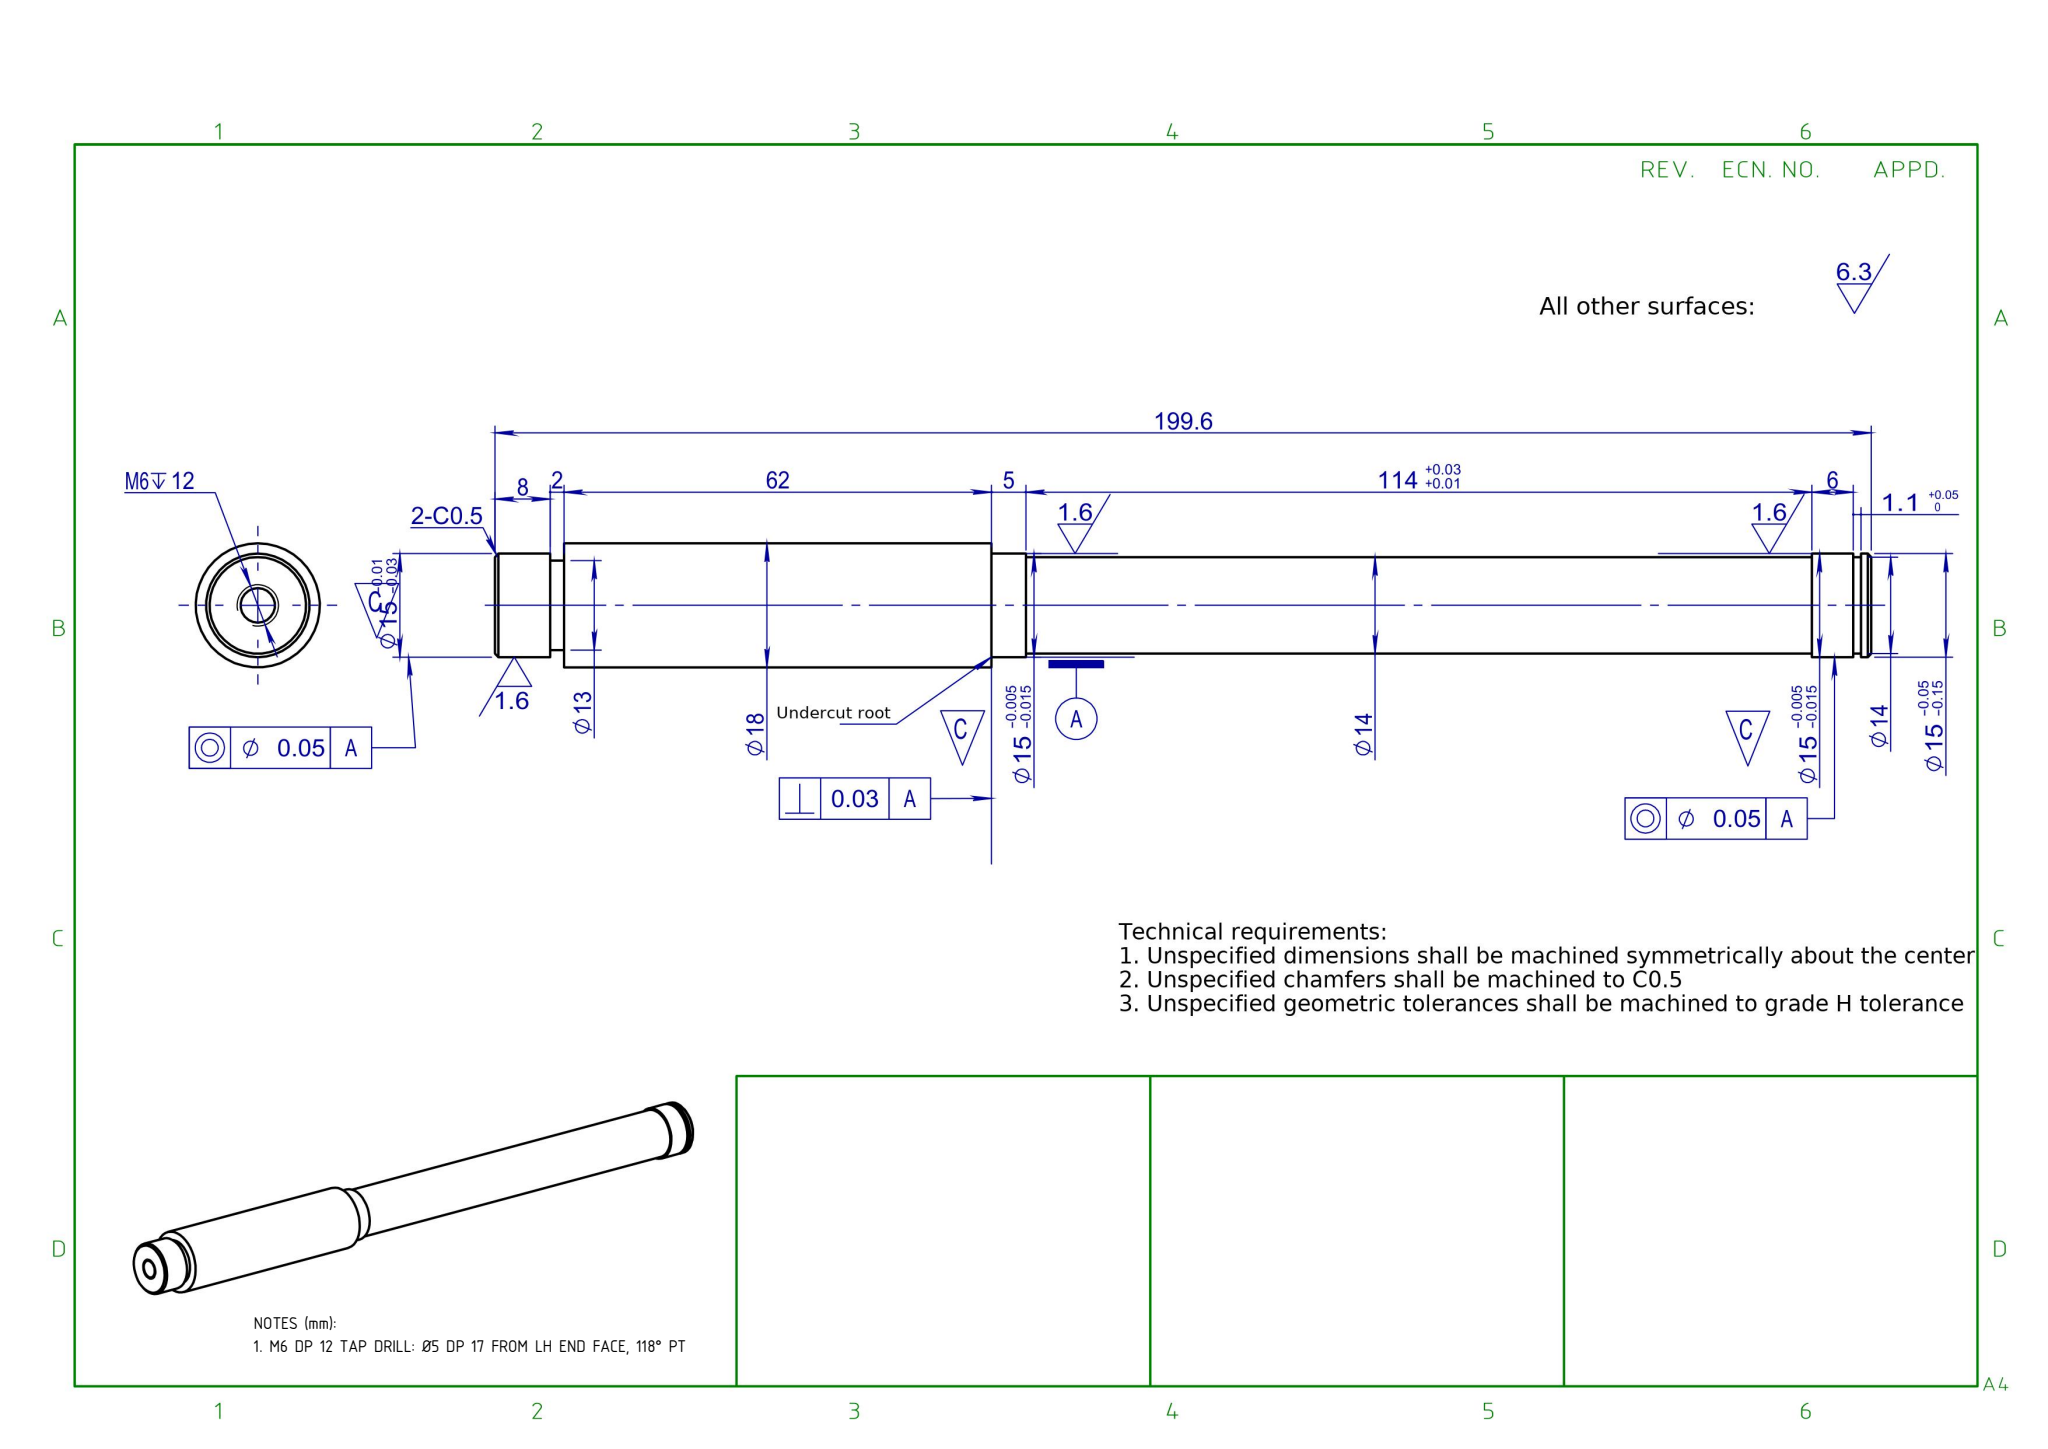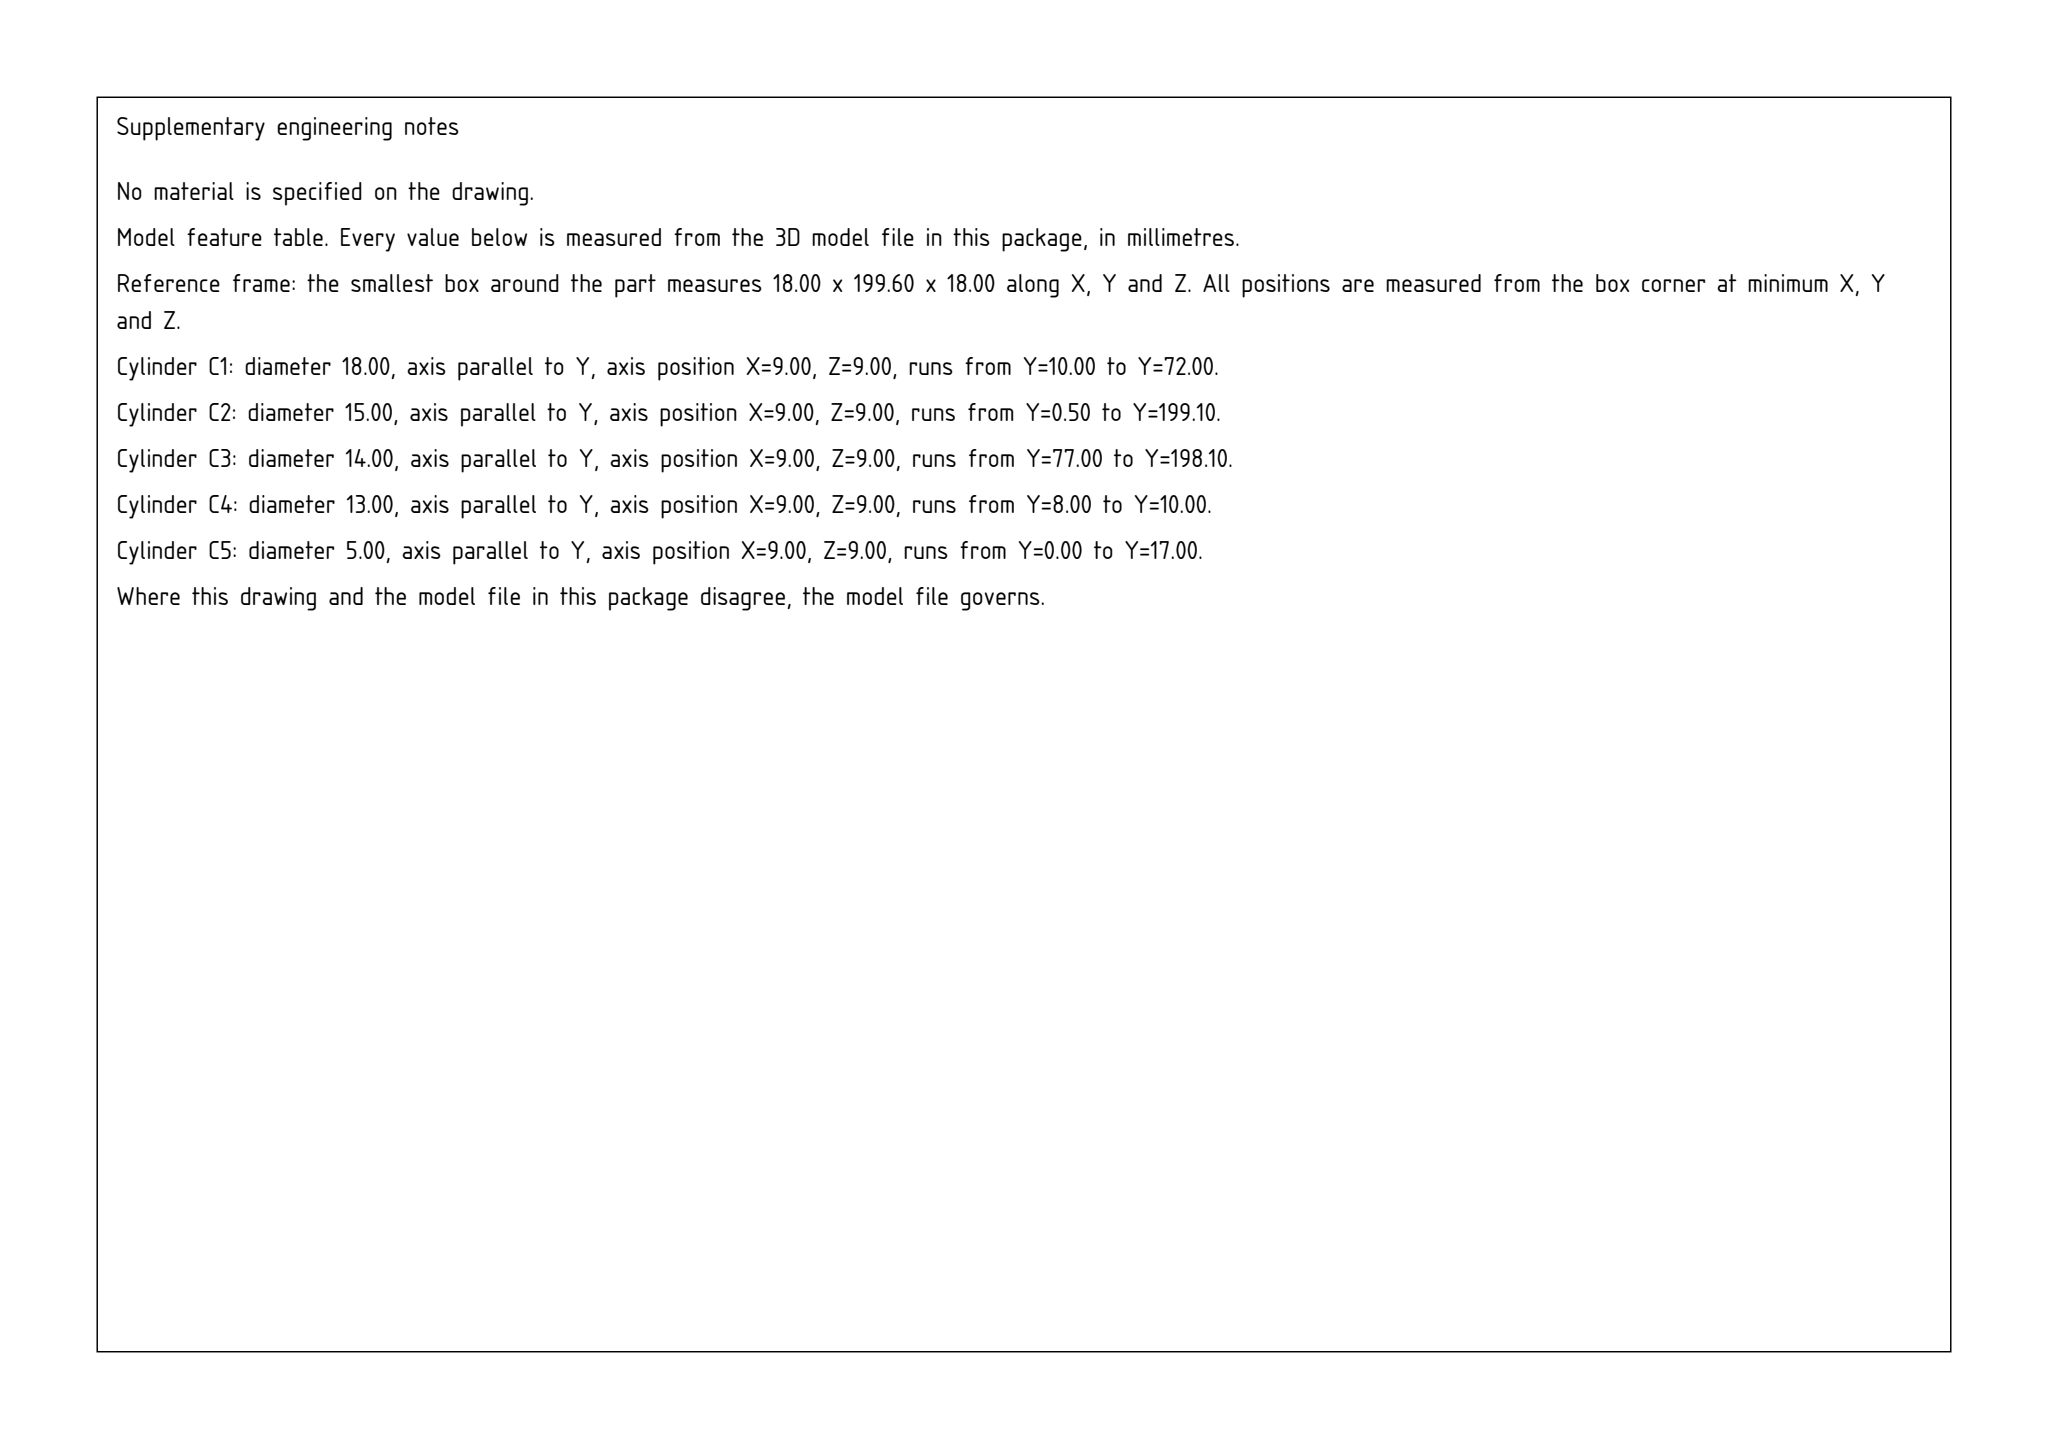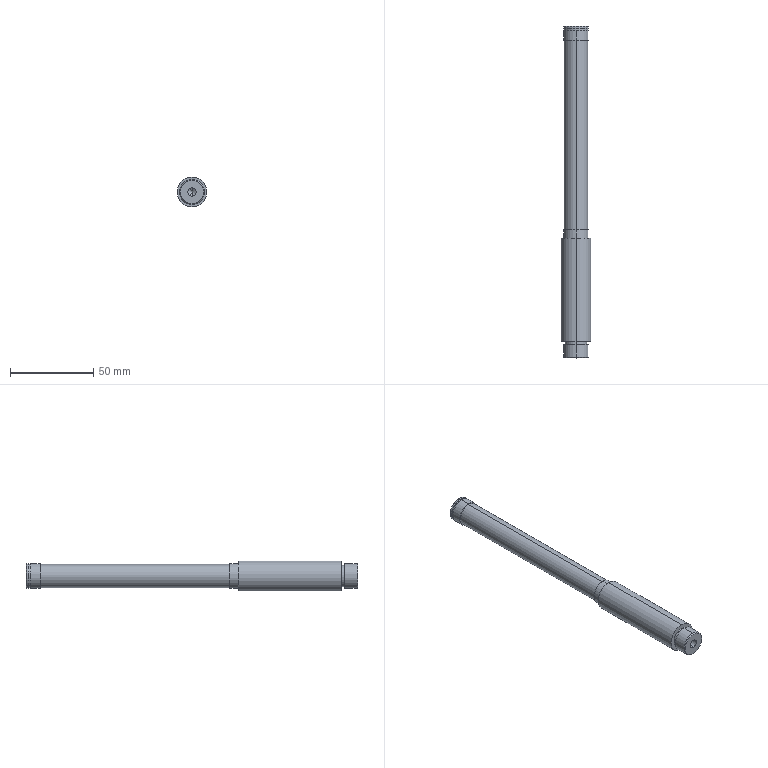Part | SolidWorks | mm | 1 solid | 33 faces | box 18 x 199.6 x 18 mm | volume 37028 mm3 | cylinder 18 | plane 9 | cone 6 | commonest cylinder face diameters 15 x8 14 x4 5 x2 13 x2 18 x2
Drawing notes:
M6 DP 12 TAP DRILL: Ø5 DP 17 FROM LH END FACE, 118° PT | from the solid: cylinder dia 5.0 axis y at (9,9), length 17.0 starting at y=0 end face; cone incl angle 118° ref dia 5.0
build123d program:
from build123d import *

# Parameters (mm, degrees)
SKETCH1_R             = 7.5
EXTRUDE1_DEPTH        = 10
SKETCH2_R             = 9
EXTRUDE2_DEPTH        = 62
SKETCH3_R             = 7.5
EXTRUDE3_DEPTH        = 5
SKETCH4_R             = 7
EXTRUDE4_DEPTH        = 114
SKETCH5_R             = 7.5
EXTRUDE5_DEPTH        = 6
SKETCH6_R             = 7
EXTRUDE6_DEPTH        = 1.1
SKETCH7_R             = 7.5
EXTRUDE7_DEPTH        = 1.5
CHAMFER1_SIZE         = 0.5
M6_TAPPED_HOLE1_D     = 5
M6_TAPPED_HOLE1_DEPTH = 17
M6_TAPPED_HOLE1_TIP   = 1.502
SKETCH10_W            = 1
SKETCH10_H            = 2
CHAMFER2_SIZE         = 0.5


with BuildPart() as part:
    # Sketch1 → Extrude1 (new body)
    with BuildSketch(Plane(origin=(0, 0, 0), x_dir=(1, 0, 0), z_dir=(0, 1, 0))):
        with Locations(Location((0, 0, 0), (0, 0, 270))):
            Circle(SKETCH1_R)
    extrude(amount=EXTRUDE1_DEPTH)

    # Sketch2 → Extrude2 (add)
    with BuildSketch(Plane(origin=(0, 10, 0), x_dir=(1, 0, 0), z_dir=(0, 1, 0))):
        with Locations(Location((0, 0, 0), (0, 0, 270))):
            Circle(SKETCH2_R)
    extrude(amount=EXTRUDE2_DEPTH)

    # Sketch3 → Extrude3 (add)
    with BuildSketch(Plane(origin=(0, 72, 0), x_dir=(1, 0, 0), z_dir=(0, 1, 0))):
        with Locations(Location((0, 0, 0), (0, 0, 270))):
            Circle(SKETCH3_R)
    extrude(amount=EXTRUDE3_DEPTH)

    # Sketch4 → Extrude4 (add)
    with BuildSketch(Plane(origin=(0, 77, 0), x_dir=(1, 0, 0), z_dir=(0, 1, 0))):
        with Locations(Location((0, 0, 0), (0, 0, 90))):
            Circle(SKETCH4_R)
    extrude(amount=EXTRUDE4_DEPTH)

    # Sketch5 → Extrude5 (add)
    with BuildSketch(Plane(origin=(0, 191, 0), x_dir=(1, 0, 0), z_dir=(0, 1, 0))):
        with Locations(Location((0, 0, 0), (0, 0, 270))):
            Circle(SKETCH5_R)
    extrude(amount=EXTRUDE5_DEPTH)

    # Sketch6 → Extrude6 (add)
    with BuildSketch(Plane(origin=(0, 197, 0), x_dir=(1, 0, 0), z_dir=(0, 1, 0))):
        with Locations(Location((0, 0, 0), (0, 0, 90))):
            Circle(SKETCH6_R)
    extrude(amount=EXTRUDE6_DEPTH)

    # Sketch7 → Extrude7 (add)
    with BuildSketch(Plane(origin=(0, 198.1, 0), x_dir=(1, 0, 0), z_dir=(0, 1, 0))):
        with Locations(Location((0, 0, 0), (0, 0, 270))):
            Circle(SKETCH7_R)
    extrude(amount=EXTRUDE7_DEPTH)

    # Chamfer1
    chamfer1_edges = [part.edges().sort_by_distance(p)[0] for p in [
        (0, 199.6, -7.5),
    ]]
    chamfer(chamfer1_edges, length=CHAMFER1_SIZE)

    # M6 Tapped Hole1
    with Locations(Plane.XZ):
        with Locations((0, 0)):
            Hole(M6_TAPPED_HOLE1_D / 2, depth=M6_TAPPED_HOLE1_DEPTH)
            with Locations((0, 0, -(M6_TAPPED_HOLE1_DEPTH + M6_TAPPED_HOLE1_TIP / 2))):  # 118° drill point
                Cone(0, M6_TAPPED_HOLE1_D / 2, M6_TAPPED_HOLE1_TIP, mode=Mode.SUBTRACT)

    # Sketch10 → Revolve-Cut1 (revolve, cut)
    with BuildSketch(Plane.XY, mode=Mode.PRIVATE) as revolve_cut1_sk:
        with Locations((-7, 9)):
            Rectangle(SKETCH10_W, SKETCH10_H)
    revolve(revolve_cut1_sk.sketch.rotate(Axis((0, 0, 0), (0, 1, 0)), 270), axis=Axis((0, 0, 0), (0, 1, 0)), mode=Mode.SUBTRACT)

    # Chamfer2
    chamfer2_edges = [part.edges().sort_by_distance(p)[0] for p in [
        (0, 0, -7.5),
    ]]
    chamfer(chamfer2_edges, length=CHAMFER2_SIZE)


solid = part.part
STEP:
#1=CARTESIAN_POINT('',(0.,0.,-7.));
#2=VERTEX_POINT('',#1);
#3=CARTESIAN_POINT('',(0.,0.,7.));
#4=VERTEX_POINT('',#3);
#5=CARTESIAN_POINT('',(0.,0.,0.));
#6=DIRECTION('',(0.,-1.,0.));
#7=DIRECTION('',(0.,0.,1.));
#8=AXIS2_PLACEMENT_3D('',#5,#6,#7);
#9=CIRCLE('',#8,7.);
#10=EDGE_CURVE('',#2,#4,#9,.T.);
#11=ORIENTED_EDGE('',*,*,#10,.F.);
#12=CARTESIAN_POINT('',(0.,0.5,-7.5));
#13=VERTEX_POINT('',#12);
#14=CARTESIAN_POINT('',(0.,0.5,-7.5));
#15=DIRECTION('',(0.,0.7071,-0.7071));
#16=VECTOR('',#15,1000.);
#17=LINE('',#14,#16);
#18=EDGE_CURVE('',#2,#13,#17,.T.);
#19=ORIENTED_EDGE('',*,*,#18,.T.);
#20=CARTESIAN_POINT('',(0.,0.5,7.5));
#21=VERTEX_POINT('',#20);
#22=CARTESIAN_POINT('',(0.,0.5,0.));
#23=DIRECTION('',(0.,1.,0.));
#24=DIRECTION('',(0.,0.,1.));
#25=AXIS2_PLACEMENT_3D('',#22,#23,#24);
#26=CIRCLE('',#25,7.5);
#27=EDGE_CURVE('',#21,#13,#26,.T.);
#28=ORIENTED_EDGE('',*,*,#27,.F.);
#29=CARTESIAN_POINT('',(0.,0.5,7.5));
#30=DIRECTION('',(0.,0.7071,0.7071));
#31=VECTOR('',#30,1000.);
#32=LINE('',#29,#31);
#33=EDGE_CURVE('',#4,#21,#32,.T.);
#34=ORIENTED_EDGE('',*,*,#33,.F.);
#35=EDGE_LOOP('',(#11,#19,#28,#34));
#36=FACE_OUTER_BOUND('',#35,.T.);
#37=CARTESIAN_POINT('',(0.,0.5,0.));
#38=DIRECTION('',(0.,1.,0.));
#39=DIRECTION('',(0.,0.,1.));
#40=AXIS2_PLACEMENT_3D('',#37,#38,#39);
#41=CONICAL_SURFACE('',#40,7.5,0.7854);
#42=ADVANCED_FACE('',(#36),#41,.T.);
#43=CARTESIAN_POINT('',(0.,8.,-7.5));
#44=VERTEX_POINT('',#43);
#45=CARTESIAN_POINT('',(0.,8.,7.5));
#46=VERTEX_POINT('',#45);
#47=CARTESIAN_POINT('',(0.,8.,0.));
#48=DIRECTION('',(0.,-1.,0.));
#49=DIRECTION('',(0.,0.,-1.));
#50=AXIS2_PLACEMENT_3D('',#47,#48,#49);
#51=CIRCLE('',#50,7.5);
#52=EDGE_CURVE('',#44,#46,#51,.T.);
#53=ORIENTED_EDGE('',*,*,#52,.T.);
#54=CARTESIAN_POINT('',(0.,10.,7.5));
#55=DIRECTION('',(0.,-1.,0.));
#56=VECTOR('',#55,1000.);
#57=LINE('',#54,#56);
#58=EDGE_CURVE('',#46,#21,#57,.T.);
#59=ORIENTED_EDGE('',*,*,#58,.T.);
#60=ORIENTED_EDGE('',*,*,#27,.T.);
#61=CARTESIAN_POINT('',(0.,10.,-7.5));
#62=DIRECTION('',(0.,-1.,0.));
#63=VECTOR('',#62,1000.);
#64=LINE('',#61,#63);
#65=EDGE_CURVE('',#44,#13,#64,.T.);
#66=ORIENTED_EDGE('',*,*,#65,.F.);
#67=EDGE_LOOP('',(#53,#59,#60,#66));
#68=FACE_OUTER_BOUND('',#67,.T.);
#69=CARTESIAN_POINT('',(0.,10.,0.));
#70=DIRECTION('',(0.,-1.,0.));
#71=DIRECTION('',(0.,0.,-1.));
#72=AXIS2_PLACEMENT_3D('',#69,#70,#71);
#73=CYLINDRICAL_SURFACE('',#72,7.5);
#74=ADVANCED_FACE('',(#68),#73,.T.);
#75=CARTESIAN_POINT('',(0.,17.,2.5));
#76=VERTEX_POINT('',#75);
#77=CARTESIAN_POINT('',(0.,17.,-2.5));
#78=VERTEX_POINT('',#77);
#79=CARTESIAN_POINT('',(0.,17.,0.));
#80=DIRECTION('',(0.,-1.,0.));
#81=DIRECTION('',(0.,0.,-1.));
#82=AXIS2_PLACEMENT_3D('',#79,#80,#81);
#83=CIRCLE('',#82,2.5);
#84=EDGE_CURVE('',#76,#78,#83,.T.);
#85=ORIENTED_EDGE('',*,*,#84,.F.);
#86=CARTESIAN_POINT('',(0.,-0.,2.5));
#87=VERTEX_POINT('',#86);
#88=CARTESIAN_POINT('',(0.,0.,2.5));
#89=DIRECTION('',(0.,-1.,0.));
#90=VECTOR('',#89,1000.);
#91=LINE('',#88,#90);
#92=EDGE_CURVE('',#76,#87,#91,.T.);
#93=ORIENTED_EDGE('',*,*,#92,.T.);
#94=CARTESIAN_POINT('',(0.,-0.,-2.5));
#95=VERTEX_POINT('',#94);
#96=CARTESIAN_POINT('',(0.,-0.,0.));
#97=DIRECTION('',(0.,-1.,0.));
#98=DIRECTION('',(0.,0.,-1.));
#99=AXIS2_PLACEMENT_3D('',#96,#97,#98);
#100=CIRCLE('',#99,2.5);
#101=EDGE_CURVE('',#87,#95,#100,.T.);
#102=ORIENTED_EDGE('',*,*,#101,.T.);
#103=CARTESIAN_POINT('',(0.,0.,-2.5));
#104=DIRECTION('',(0.,-1.,0.));
#105=VECTOR('',#104,1000.);
#106=LINE('',#103,#105);
#107=EDGE_CURVE('',#78,#95,#106,.T.);
#108=ORIENTED_EDGE('',*,*,#107,.F.);
#109=EDGE_LOOP('',(#85,#93,#102,#108));
#110=FACE_OUTER_BOUND('',#109,.T.);
#111=CARTESIAN_POINT('',(0.,0.,0.));
#112=DIRECTION('',(0.,-1.,0.));
#113=DIRECTION('',(0.,0.,-1.));
#114=AXIS2_PLACEMENT_3D('',#111,#112,#113);
#115=CYLINDRICAL_SURFACE('',#114,2.5);
#116=ADVANCED_FACE('',(#110),#115,.F.);
#117=CARTESIAN_POINT('',(-0.,18.502,0.));
#118=VERTEX_POINT('',#117);
#119=CARTESIAN_POINT('',(0.,17.,-2.5));
#120=DIRECTION('',(0.,-0.515,-0.8572));
#121=VECTOR('',#120,1000.);
#122=LINE('',#119,#121);
#123=EDGE_CURVE('',#118,#78,#122,.T.);
#124=ORIENTED_EDGE('',*,*,#123,.F.);
#125=CARTESIAN_POINT('',(0.,17.,2.5));
#126=DIRECTION('',(0.,-0.515,0.8572));
#127=VECTOR('',#126,1000.);
#128=LINE('',#125,#127);
#129=EDGE_CURVE('',#118,#76,#128,.T.);
#130=ORIENTED_EDGE('',*,*,#129,.T.);
#131=ORIENTED_EDGE('',*,*,#84,.T.);
#132=EDGE_LOOP('',(#124,#130,#131));
#133=FACE_OUTER_BOUND('',#132,.T.);
#134=CARTESIAN_POINT('',(0.,17.,0.));
#135=DIRECTION('',(0.,-1.,0.));
#136=DIRECTION('',(0.,0.,-1.));
#137=AXIS2_PLACEMENT_3D('',#134,#135,#136);
#138=CONICAL_SURFACE('',#137,2.5,1.03);
#139=ADVANCED_FACE('',(#133),#138,.F.);
#140=CARTESIAN_POINT('',(0.,10.,-6.5));
#141=VERTEX_POINT('',#140);
#142=CARTESIAN_POINT('',(0.,10.,6.5));
#143=VERTEX_POINT('',#142);
#144=CARTESIAN_POINT('',(0.,10.,0.));
#145=DIRECTION('',(0.,-1.,0.));
#146=DIRECTION('',(0.,0.,-1.));
#147=AXIS2_PLACEMENT_3D('',#144,#145,#146);
#148=CIRCLE('',#147,6.5);
#149=EDGE_CURVE('',#141,#143,#148,.T.);
#150=ORIENTED_EDGE('',*,*,#149,.T.);
#151=CARTESIAN_POINT('',(0.,8.,6.5));
#152=VERTEX_POINT('',#151);
#153=CARTESIAN_POINT('',(0.,0.,6.5));
#154=DIRECTION('',(0.,-1.,0.));
#155=VECTOR('',#154,1000.);
#156=LINE('',#153,#155);
#157=EDGE_CURVE('',#143,#152,#156,.T.);
#158=ORIENTED_EDGE('',*,*,#157,.T.);
#159=CARTESIAN_POINT('',(0.,8.,-6.5));
#160=VERTEX_POINT('',#159);
#161=CARTESIAN_POINT('',(0.,8.,0.));
#162=DIRECTION('',(0.,-1.,0.));
#163=DIRECTION('',(0.,0.,-1.));
#164=AXIS2_PLACEMENT_3D('',#161,#162,#163);
#165=CIRCLE('',#164,6.5);
#166=EDGE_CURVE('',#160,#152,#165,.T.);
#167=ORIENTED_EDGE('',*,*,#166,.F.);
#168=CARTESIAN_POINT('',(0.,0.,-6.5));
#169=DIRECTION('',(0.,-1.,0.));
#170=VECTOR('',#169,1000.);
#171=LINE('',#168,#170);
#172=EDGE_CURVE('',#141,#160,#171,.T.);
#173=ORIENTED_EDGE('',*,*,#172,.F.);
#174=EDGE_LOOP('',(#150,#158,#167,#173));
#175=FACE_OUTER_BOUND('',#174,.T.);
#176=CARTESIAN_POINT('',(0.,0.,0.));
#177=DIRECTION('',(0.,-1.,0.));
#178=DIRECTION('',(0.,0.,-1.));
#179=AXIS2_PLACEMENT_3D('',#176,#177,#178);
#180=CYLINDRICAL_SURFACE('',#179,6.5);
#181=ADVANCED_FACE('',(#175),#180,.T.);
#182=CARTESIAN_POINT('',(0.,199.6,7.));
#183=VERTEX_POINT('',#182);
#184=CARTESIAN_POINT('',(0.,199.6,-7.));
#185=VERTEX_POINT('',#184);
#186=CARTESIAN_POINT('',(0.,199.6,0.));
#187=DIRECTION('',(0.,1.,0.));
#188=DIRECTION('',(0.,0.,1.));
#189=AXIS2_PLACEMENT_3D('',#186,#187,#188);
#190=CIRCLE('',#189,7.);
#191=EDGE_CURVE('',#183,#185,#190,.T.);
#192=ORIENTED_EDGE('',*,*,#191,.F.);
#193=CARTESIAN_POINT('',(0.,199.1,7.5));
#194=VERTEX_POINT('',#193);
#195=CARTESIAN_POINT('',(0.,199.6,7.));
#196=DIRECTION('',(0.,-0.7071,0.7071));
#197=VECTOR('',#196,1000.);
#198=LINE('',#195,#197);
#199=EDGE_CURVE('',#183,#194,#198,.T.);
#200=ORIENTED_EDGE('',*,*,#199,.T.);
#201=CARTESIAN_POINT('',(0.,199.1,-7.5));
#202=VERTEX_POINT('',#201);
#203=CARTESIAN_POINT('',(0.,199.1,0.));
#204=DIRECTION('',(0.,-1.,0.));
#205=DIRECTION('',(0.,0.,1.));
#206=AXIS2_PLACEMENT_3D('',#203,#204,#205);
#207=CIRCLE('',#206,7.5);
#208=EDGE_CURVE('',#202,#194,#207,.T.);
#209=ORIENTED_EDGE('',*,*,#208,.F.);
#210=CARTESIAN_POINT('',(0.,199.6,-7.));
#211=DIRECTION('',(0.,-0.7071,-0.7071));
#212=VECTOR('',#211,1000.);
#213=LINE('',#210,#212);
#214=EDGE_CURVE('',#185,#202,#213,.T.);
#215=ORIENTED_EDGE('',*,*,#214,.F.);
#216=EDGE_LOOP('',(#192,#200,#209,#215));
#217=FACE_OUTER_BOUND('',#216,.T.);
#218=CARTESIAN_POINT('',(0.,199.6,0.));
#219=DIRECTION('',(0.,-1.,0.));
#220=DIRECTION('',(0.,0.,-1.));
#221=AXIS2_PLACEMENT_3D('',#218,#219,#220);
#222=CONICAL_SURFACE('',#221,7.,0.7854);
#223=ADVANCED_FACE('',(#217),#222,.T.);
#224=ORIENTED_EDGE('',*,*,#208,.T.);
#225=CARTESIAN_POINT('',(0.,198.1,7.5));
#226=VERTEX_POINT('',#225);
#227=CARTESIAN_POINT('',(0.,199.6,7.5));
#228=DIRECTION('',(0.,-1.,0.));
#229=VECTOR('',#228,1000.);
#230=LINE('',#227,#229);
#231=EDGE_CURVE('',#194,#226,#230,.T.);
#232=ORIENTED_EDGE('',*,*,#231,.T.);
#233=CARTESIAN_POINT('',(0.,198.1,-7.5));
#234=VERTEX_POINT('',#233);
#235=CARTESIAN_POINT('',(0.,198.1,0.));
#236=DIRECTION('',(0.,1.,0.));
#237=DIRECTION('',(0.,0.,1.));
#238=AXIS2_PLACEMENT_3D('',#235,#236,#237);
#239=CIRCLE('',#238,7.5);
#240=EDGE_CURVE('',#226,#234,#239,.T.);
#241=ORIENTED_EDGE('',*,*,#240,.T.);
#242=CARTESIAN_POINT('',(0.,199.6,-7.5));
#243=DIRECTION('',(0.,-1.,0.));
#244=VECTOR('',#243,1000.);
#245=LINE('',#242,#244);
#246=EDGE_CURVE('',#202,#234,#245,.T.);
#247=ORIENTED_EDGE('',*,*,#246,.F.);
#248=EDGE_LOOP('',(#224,#232,#241,#247));
#249=FACE_OUTER_BOUND('',#248,.T.);
#250=CARTESIAN_POINT('',(0.,199.6,0.));
#251=DIRECTION('',(0.,-1.,0.));
#252=DIRECTION('',(0.,0.,-1.));
#253=AXIS2_PLACEMENT_3D('',#250,#251,#252);
#254=CYLINDRICAL_SURFACE('',#253,7.5);
#255=ADVANCED_FACE('',(#249),#254,.T.);
#256=CARTESIAN_POINT('',(0.,198.1,7.));
#257=VERTEX_POINT('',#256);
#258=CARTESIAN_POINT('',(0.,198.1,-7.));
#259=VERTEX_POINT('',#258);
#260=CARTESIAN_POINT('',(0.,198.1,0.));
#261=DIRECTION('',(0.,1.,0.));
#262=DIRECTION('',(0.,0.,1.));
#263=AXIS2_PLACEMENT_3D('',#260,#261,#262);
#264=CIRCLE('',#263,7.);
#265=EDGE_CURVE('',#257,#259,#264,.T.);
#266=ORIENTED_EDGE('',*,*,#265,.F.);
#267=CARTESIAN_POINT('',(0.,197.,7.));
#268=VERTEX_POINT('',#267);
#269=CARTESIAN_POINT('',(0.,198.1,7.));
#270=DIRECTION('',(0.,-1.,0.));
#271=VECTOR('',#270,1000.);
#272=LINE('',#269,#271);
#273=EDGE_CURVE('',#257,#268,#272,.T.);
#274=ORIENTED_EDGE('',*,*,#273,.T.);
#275=CARTESIAN_POINT('',(0.,197.,-7.));
#276=VERTEX_POINT('',#275);
#277=CARTESIAN_POINT('',(0.,197.,0.));
#278=DIRECTION('',(0.,1.,0.));
#279=DIRECTION('',(0.,0.,1.));
#280=AXIS2_PLACEMENT_3D('',#277,#278,#279);
#281=CIRCLE('',#280,7.);
#282=EDGE_CURVE('',#268,#276,#281,.T.);
#283=ORIENTED_EDGE('',*,*,#282,.T.);
#284=CARTESIAN_POINT('',(0.,198.1,-7.));
#285=DIRECTION('',(0.,-1.,0.));
#286=VECTOR('',#285,1000.);
#287=LINE('',#284,#286);
#288=EDGE_CURVE('',#259,#276,#287,.T.);
#289=ORIENTED_EDGE('',*,*,#288,.F.);
#290=EDGE_LOOP('',(#266,#274,#283,#289));
#291=FACE_OUTER_BOUND('',#290,.T.);
#292=CARTESIAN_POINT('',(0.,198.1,0.));
#293=DIRECTION('',(0.,-1.,0.));
#294=DIRECTION('',(0.,0.,-1.));
#295=AXIS2_PLACEMENT_3D('',#292,#293,#294);
#296=CYLINDRICAL_SURFACE('',#295,7.);
#297=ADVANCED_FACE('',(#291),#296,.T.);
#298=CARTESIAN_POINT('',(0.,197.,7.5));
#299=VERTEX_POINT('',#298);
#300=CARTESIAN_POINT('',(0.,197.,-7.5));
#301=VERTEX_POINT('',#300);
#302=CARTESIAN_POINT('',(0.,197.,0.));
#303=DIRECTION('',(0.,1.,0.));
#304=DIRECTION('',(0.,0.,1.));
#305=AXIS2_PLACEMENT_3D('',#302,#303,#304);
#306=CIRCLE('',#305,7.5);
#307=EDGE_CURVE('',#299,#301,#306,.T.);
#308=ORIENTED_EDGE('',*,*,#307,.F.);
#309=CARTESIAN_POINT('',(0.,191.,7.5));
#310=VERTEX_POINT('',#309);
#311=CARTESIAN_POINT('',(0.,197.,7.5));
#312=DIRECTION('',(0.,-1.,0.));
#313=VECTOR('',#312,1000.);
#314=LINE('',#311,#313);
#315=EDGE_CURVE('',#299,#310,#314,.T.);
#316=ORIENTED_EDGE('',*,*,#315,.T.);
#317=CARTESIAN_POINT('',(0.,191.,-7.5));
#318=VERTEX_POINT('',#317);
#319=CARTESIAN_POINT('',(0.,191.,0.));
#320=DIRECTION('',(0.,1.,0.));
#321=DIRECTION('',(0.,0.,1.));
#322=AXIS2_PLACEMENT_3D('',#319,#320,#321);
#323=CIRCLE('',#322,7.5);
#324=EDGE_CURVE('',#310,#318,#323,.T.);
#325=ORIENTED_EDGE('',*,*,#324,.T.);
#326=CARTESIAN_POINT('',(0.,197.,-7.5));
#327=DIRECTION('',(0.,-1.,0.));
#328=VECTOR('',#327,1000.);
#329=LINE('',#326,#328);
#330=EDGE_CURVE('',#301,#318,#329,.T.);
#331=ORIENTED_EDGE('',*,*,#330,.F.);
#332=EDGE_LOOP('',(#308,#316,#325,#331));
#333=FACE_OUTER_BOUND('',#332,.T.);
#334=CARTESIAN_POINT('',(0.,197.,0.));
#335=DIRECTION('',(0.,-1.,0.));
#336=DIRECTION('',(0.,0.,-1.));
#337=AXIS2_PLACEMENT_3D('',#334,#335,#336);
#338=CYLINDRICAL_SURFACE('',#337,7.5);
#339=ADVANCED_FACE('',(#333),#338,.T.);
#340=CARTESIAN_POINT('',(0.,191.,7.));
#341=VERTEX_POINT('',#340);
#342=CARTESIAN_POINT('',(0.,191.,-7.));
#343=VERTEX_POINT('',#342);
#344=CARTESIAN_POINT('',(0.,191.,0.));
#345=DIRECTION('',(0.,1.,0.));
#346=DIRECTION('',(0.,0.,1.));
#347=AXIS2_PLACEMENT_3D('',#344,#345,#346);
#348=CIRCLE('',#347,7.);
#349=EDGE_CURVE('',#341,#343,#348,.T.);
#350=ORIENTED_EDGE('',*,*,#349,.F.);
#351=CARTESIAN_POINT('',(0.,77.,7.));
#352=VERTEX_POINT('',#351);
#353=CARTESIAN_POINT('',(0.,191.,7.));
#354=DIRECTION('',(0.,-1.,0.));
#355=VECTOR('',#354,1000.);
#356=LINE('',#353,#355);
#357=EDGE_CURVE('',#341,#352,#356,.T.);
#358=ORIENTED_EDGE('',*,*,#357,.T.);
#359=CARTESIAN_POINT('',(0.,77.,-7.));
#360=VERTEX_POINT('',#359);
#361=CARTESIAN_POINT('',(0.,77.,0.));
#362=DIRECTION('',(0.,1.,0.));
#363=DIRECTION('',(0.,0.,1.));
#364=AXIS2_PLACEMENT_3D('',#361,#362,#363);
#365=CIRCLE('',#364,7.);
#366=EDGE_CURVE('',#352,#360,#365,.T.);
#367=ORIENTED_EDGE('',*,*,#366,.T.);
#368=CARTESIAN_POINT('',(0.,191.,-7.));
#369=DIRECTION('',(0.,-1.,0.));
#370=VECTOR('',#369,1000.);
#371=LINE('',#368,#370);
#372=EDGE_CURVE('',#343,#360,#371,.T.);
#373=ORIENTED_EDGE('',*,*,#372,.F.);
#374=EDGE_LOOP('',(#350,#358,#367,#373));
#375=FACE_OUTER_BOUND('',#374,.T.);
#376=CARTESIAN_POINT('',(0.,191.,0.));
#377=DIRECTION('',(0.,-1.,0.));
#378=DIRECTION('',(0.,0.,-1.));
#379=AXIS2_PLACEMENT_3D('',#376,#377,#378);
#380=CYLINDRICAL_SURFACE('',#379,7.);
#381=ADVANCED_FACE('',(#375),#380,.T.);
#382=CARTESIAN_POINT('',(0.,77.,7.5));
#383=VERTEX_POINT('',#382);
#384=CARTESIAN_POINT('',(0.,77.,-7.5));
#385=VERTEX_POINT('',#384);
#386=CARTESIAN_POINT('',(0.,77.,0.));
#387=DIRECTION('',(0.,1.,0.));
#388=DIRECTION('',(0.,0.,1.));
#389=AXIS2_PLACEMENT_3D('',#386,#387,#388);
#390=CIRCLE('',#389,7.5);
#391=EDGE_CURVE('',#383,#385,#390,.T.);
#392=ORIENTED_EDGE('',*,*,#391,.F.);
#393=CARTESIAN_POINT('',(0.,72.,7.5));
#394=VERTEX_POINT('',#393);
#395=CARTESIAN_POINT('',(0.,77.,7.5));
#396=DIRECTION('',(0.,-1.,0.));
#397=VECTOR('',#396,1000.);
#398=LINE('',#395,#397);
#399=EDGE_CURVE('',#383,#394,#398,.T.);
#400=ORIENTED_EDGE('',*,*,#399,.T.);
#401=CARTESIAN_POINT('',(0.,72.,-7.5));
#402=VERTEX_POINT('',#401);
#403=CARTESIAN_POINT('',(0.,72.,0.));
#404=DIRECTION('',(0.,1.,0.));
#405=DIRECTION('',(0.,0.,1.));
#406=AXIS2_PLACEMENT_3D('',#403,#404,#405);
#407=CIRCLE('',#406,7.5);
#408=EDGE_CURVE('',#394,#402,#407,.T.);
#409=ORIENTED_EDGE('',*,*,#408,.T.);
#410=CARTESIAN_POINT('',(0.,77.,-7.5));
#411=DIRECTION('',(0.,-1.,0.));
#412=VECTOR('',#411,1000.);
#413=LINE('',#410,#412);
#414=EDGE_CURVE('',#385,#402,#413,.T.);
#415=ORIENTED_EDGE('',*,*,#414,.F.);
#416=EDGE_LOOP('',(#392,#400,#409,#415));
#417=FACE_OUTER_BOUND('',#416,.T.);
#418=CARTESIAN_POINT('',(0.,77.,0.));
#419=DIRECTION('',(0.,-1.,0.));
#420=DIRECTION('',(0.,0.,-1.));
#421=AXIS2_PLACEMENT_3D('',#418,#419,#420);
#422=CYLINDRICAL_SURFACE('',#421,7.5);
#423=ADVANCED_FACE('',(#417),#422,.T.);
#424=CARTESIAN_POINT('',(0.,72.,9.));
#425=VERTEX_POINT('',#424);
#426=CARTESIAN_POINT('',(0.,72.,-9.));
#427=VERTEX_POINT('',#426);
#428=CARTESIAN_POINT('',(0.,72.,0.));
#429=DIRECTION('',(0.,1.,0.));
#430=DIRECTION('',(0.,0.,1.));
#431=AXIS2_PLACEMENT_3D('',#428,#429,#430);
#432=CIRCLE('',#431,9.);
#433=EDGE_CURVE('',#425,#427,#432,.T.);
#434=ORIENTED_EDGE('',*,*,#433,.F.);
#435=CARTESIAN_POINT('',(0.,10.,9.));
#436=VERTEX_POINT('',#435);
#437=CARTESIAN_POINT('',(0.,72.,9.));
#438=DIRECTION('',(0.,-1.,0.));
#439=VECTOR('',#438,1000.);
#440=LINE('',#437,#439);
#441=EDGE_CURVE('',#425,#436,#440,.T.);
#442=ORIENTED_EDGE('',*,*,#441,.T.);
#443=CARTESIAN_POINT('',(0.,10.,-9.));
#444=VERTEX_POINT('',#443);
#445=CARTESIAN_POINT('',(0.,10.,0.));
#446=DIRECTION('',(0.,1.,0.));
#447=DIRECTION('',(0.,0.,1.));
#448=AXIS2_PLACEMENT_3D('',#445,#446,#447);
#449=CIRCLE('',#448,9.);
#450=EDGE_CURVE('',#436,#444,#449,.T.);
#451=ORIENTED_EDGE('',*,*,#450,.T.);
#452=CARTESIAN_POINT('',(0.,72.,-9.));
#453=DIRECTION('',(0.,-1.,0.));
#454=VECTOR('',#453,1000.);
#455=LINE('',#452,#454);
#456=EDGE_CURVE('',#427,#444,#455,.T.);
#457=ORIENTED_EDGE('',*,*,#456,.F.);
#458=EDGE_LOOP('',(#434,#442,#451,#457));
#459=FACE_OUTER_BOUND('',#458,.T.);
#460=CARTESIAN_POINT('',(0.,72.,0.));
#461=DIRECTION('',(0.,-1.,0.));
#462=DIRECTION('',(0.,0.,-1.));
#463=AXIS2_PLACEMENT_3D('',#460,#461,#462);
#464=CYLINDRICAL_SURFACE('',#463,9.);
#465=ADVANCED_FACE('',(#459),#464,.T.);
#466=CARTESIAN_POINT('',(0.,197.,0.));
#467=DIRECTION('',(0.,1.,0.));
#468=DIRECTION('',(0.,0.,1.));
#469=AXIS2_PLACEMENT_3D('',#466,#467,#468);
#470=CIRCLE('',#469,7.5);
#471=EDGE_CURVE('',#301,#299,#470,.T.);
#472=ORIENTED_EDGE('',*,*,#471,.T.);
#473=ORIENTED_EDGE('',*,*,#307,.T.);
#474=EDGE_LOOP('',(#472,#473));
#475=FACE_OUTER_BOUND('',#474,.T.);
#476=CARTESIAN_POINT('',(0.,197.,0.));
#477=DIRECTION('',(0.,1.,0.));
#478=DIRECTION('',(0.,0.,1.));
#479=AXIS2_PLACEMENT_3D('',#476,#477,#478);
#480=CIRCLE('',#479,7.);
#481=EDGE_CURVE('',#276,#268,#480,.T.);
#482=ORIENTED_EDGE('',*,*,#481,.F.);
#483=ORIENTED_EDGE('',*,*,#282,.F.);
#484=EDGE_LOOP('',(#482,#483));
#485=FACE_BOUND('',#484,.T.);
#486=CARTESIAN_POINT('',(0.,197.,0.));
#487=DIRECTION('',(0.,1.,0.));
#488=DIRECTION('',(0.,0.,1.));
#489=AXIS2_PLACEMENT_3D('',#486,#487,#488);
#490=PLANE('',#489);
#491=ADVANCED_FACE('',(#475,#485),#490,.T.);
#492=CARTESIAN_POINT('',(0.,77.,0.));
#493=DIRECTION('',(0.,1.,0.));
#494=DIRECTION('',(0.,0.,1.));
#495=AXIS2_PLACEMENT_3D('',#492,#493,#494);
#496=CIRCLE('',#495,7.5);
#497=EDGE_CURVE('',#385,#383,#496,.T.);
#498=ORIENTED_EDGE('',*,*,#497,.T.);
#499=ORIENTED_EDGE('',*,*,#391,.T.);
#500=EDGE_LOOP('',(#498,#499));
#501=FACE_OUTER_BOUND('',#500,.T.);
#502=CARTESIAN_POINT('',(0.,77.,0.));
#503=DIRECTION('',(0.,1.,0.));
#504=DIRECTION('',(0.,0.,1.));
#505=AXIS2_PLACEMENT_3D('',#502,#503,#504);
#506=CIRCLE('',#505,7.);
#507=EDGE_CURVE('',#360,#352,#506,.T.);
#508=ORIENTED_EDGE('',*,*,#507,.F.);
#509=ORIENTED_EDGE('',*,*,#366,.F.);
#510=EDGE_LOOP('',(#508,#509));
#511=FACE_BOUND('',#510,.T.);
#512=CARTESIAN_POINT('',(0.,77.,0.));
#513=DIRECTION('',(0.,1.,0.));
#514=DIRECTION('',(0.,0.,1.));
#515=AXIS2_PLACEMENT_3D('',#512,#513,#514);
#516=PLANE('',#515);
#517=ADVANCED_FACE('',(#501,#511),#516,.T.);
#518=CARTESIAN_POINT('',(0.,72.,0.));
#519=DIRECTION('',(0.,1.,0.));
#520=DIRECTION('',(0.,0.,1.));
#521=AXIS2_PLACEMENT_3D('',#518,#519,#520);
#522=CIRCLE('',#521,9.);
#523=EDGE_CURVE('',#427,#425,#522,.T.);
#524=ORIENTED_EDGE('',*,*,#523,.T.);
#525=ORIENTED_EDGE('',*,*,#433,.T.);
#526=EDGE_LOOP('',(#524,#525));
#527=FACE_OUTER_BOUND('',#526,.T.);
#528=CARTESIAN_POINT('',(0.,72.,0.));
#529=DIRECTION('',(0.,1.,0.));
#530=DIRECTION('',(0.,0.,1.));
#531=AXIS2_PLACEMENT_3D('',#528,#529,#530);
#532=CIRCLE('',#531,7.5);
#533=EDGE_CURVE('',#402,#394,#532,.T.);
#534=ORIENTED_EDGE('',*,*,#533,.F.);
#535=ORIENTED_EDGE('',*,*,#408,.F.);
#536=EDGE_LOOP('',(#534,#535));
#537=FACE_BOUND('',#536,.T.);
#538=CARTESIAN_POINT('',(0.,72.,0.));
#539=DIRECTION('',(0.,1.,0.));
#540=DIRECTION('',(0.,0.,1.));
#541=AXIS2_PLACEMENT_3D('',#538,#539,#540);
#542=PLANE('',#541);
#543=ADVANCED_FACE('',(#527,#537),#542,.T.);
#544=CARTESIAN_POINT('',(0.,10.,0.));
#545=DIRECTION('',(0.,1.,0.));
#546=DIRECTION('',(0.,0.,1.));
#547=AXIS2_PLACEMENT_3D('',#544,#545,#546);
#548=CIRCLE('',#547,9.);
#549=EDGE_CURVE('',#444,#436,#548,.T.);
#550=ORIENTED_EDGE('',*,*,#549,.F.);
#551=ORIENTED_EDGE('',*,*,#450,.F.);
#552=EDGE_LOOP('',(#550,#551));
#553=FACE_OUTER_BOUND('',#552,.T.);
#554=ORIENTED_EDGE('',*,*,#149,.F.);
#555=CARTESIAN_POINT('',(0.,10.,0.));
#556=DIRECTION('',(0.,-1.,0.));
#557=DIRECTION('',(0.,0.,-1.));
#558=AXIS2_PLACEMENT_3D('',#555,#556,#557);
#559=CIRCLE('',#558,6.5);
#560=EDGE_CURVE('',#143,#141,#559,.T.);
#561=ORIENTED_EDGE('',*,*,#560,.F.);
#562=EDGE_LOOP('',(#554,#561));
#563=FACE_BOUND('',#562,.T.);
#564=CARTESIAN_POINT('',(0.,10.,0.));
#565=DIRECTION('',(0.,1.,0.));
#566=DIRECTION('',(0.,0.,1.));
#567=AXIS2_PLACEMENT_3D('',#564,#565,#566);
#568=PLANE('',#567);
#569=ADVANCED_FACE('',(#553,#563),#568,.F.);
#570=ORIENTED_EDGE('',*,*,#441,.F.);
#571=ORIENTED_EDGE('',*,*,#523,.F.);
#572=ORIENTED_EDGE('',*,*,#456,.T.);
#573=ORIENTED_EDGE('',*,*,#549,.T.);
#574=EDGE_LOOP('',(#570,#571,#572,#573));
#575=FACE_OUTER_BOUND('',#574,.T.);
#576=CARTESIAN_POINT('',(0.,72.,0.));
#577=DIRECTION('',(0.,-1.,0.));
#578=DIRECTION('',(0.,0.,-1.));
#579=AXIS2_PLACEMENT_3D('',#576,#577,#578);
#580=CYLINDRICAL_SURFACE('',#579,9.);
#581=ADVANCED_FACE('',(#575),#580,.T.);
#582=ORIENTED_EDGE('',*,*,#399,.F.);
#583=ORIENTED_EDGE('',*,*,#497,.F.);
#584=ORIENTED_EDGE('',*,*,#414,.T.);
#585=ORIENTED_EDGE('',*,*,#533,.T.);
#586=EDGE_LOOP('',(#582,#583,#584,#585));
#587=FACE_OUTER_BOUND('',#586,.T.);
#588=CARTESIAN_POINT('',(0.,77.,0.));
#589=DIRECTION('',(0.,-1.,0.));
#590=DIRECTION('',(0.,0.,-1.));
#591=AXIS2_PLACEMENT_3D('',#588,#589,#590);
#592=CYLINDRICAL_SURFACE('',#591,7.5);
#593=ADVANCED_FACE('',(#587),#592,.T.);
#594=ORIENTED_EDGE('',*,*,#357,.F.);
#595=CARTESIAN_POINT('',(0.,191.,0.));
#596=DIRECTION('',(0.,1.,0.));
#597=DIRECTION('',(0.,0.,1.));
#598=AXIS2_PLACEMENT_3D('',#595,#596,#597);
#599=CIRCLE('',#598,7.);
#600=EDGE_CURVE('',#343,#341,#599,.T.);
#601=ORIENTED_EDGE('',*,*,#600,.F.);
#602=ORIENTED_EDGE('',*,*,#372,.T.);
#603=ORIENTED_EDGE('',*,*,#507,.T.);
#604=EDGE_LOOP('',(#594,#601,#602,#603));
#605=FACE_OUTER_BOUND('',#604,.T.);
#606=CARTESIAN_POINT('',(0.,191.,0.));
#607=DIRECTION('',(0.,-1.,0.));
#608=DIRECTION('',(0.,0.,-1.));
#609=AXIS2_PLACEMENT_3D('',#606,#607,#608);
#610=CYLINDRICAL_SURFACE('',#609,7.);
#611=ADVANCED_FACE('',(#605),#610,.T.);
#612=CARTESIAN_POINT('',(0.,191.,0.));
#613=DIRECTION('',(0.,1.,0.));
#614=DIRECTION('',(0.,0.,1.));
#615=AXIS2_PLACEMENT_3D('',#612,#613,#614);
#616=CIRCLE('',#615,7.5);
#617=EDGE_CURVE('',#318,#310,#616,.T.);
#618=ORIENTED_EDGE('',*,*,#617,.F.);
#619=ORIENTED_EDGE('',*,*,#324,.F.);
#620=EDGE_LOOP('',(#618,#619));
#621=FACE_OUTER_BOUND('',#620,.T.);
#622=ORIENTED_EDGE('',*,*,#600,.T.);
#623=ORIENTED_EDGE('',*,*,#349,.T.);
#624=EDGE_LOOP('',(#622,#623));
#625=FACE_BOUND('',#624,.T.);
#626=CARTESIAN_POINT('',(0.,191.,0.));
#627=DIRECTION('',(0.,1.,0.));
#628=DIRECTION('',(0.,0.,1.));
#629=AXIS2_PLACEMENT_3D('',#626,#627,#628);
#630=PLANE('',#629);
#631=ADVANCED_FACE('',(#621,#625),#630,.F.);
#632=ORIENTED_EDGE('',*,*,#315,.F.);
#633=ORIENTED_EDGE('',*,*,#471,.F.);
#634=ORIENTED_EDGE('',*,*,#330,.T.);
#635=ORIENTED_EDGE('',*,*,#617,.T.);
#636=EDGE_LOOP('',(#632,#633,#634,#635));
#637=FACE_OUTER_BOUND('',#636,.T.);
#638=CARTESIAN_POINT('',(0.,197.,0.));
#639=DIRECTION('',(0.,-1.,0.));
#640=DIRECTION('',(0.,0.,-1.));
#641=AXIS2_PLACEMENT_3D('',#638,#639,#640);
#642=CYLINDRICAL_SURFACE('',#641,7.5);
#643=ADVANCED_FACE('',(#637),#642,.T.);
#644=ORIENTED_EDGE('',*,*,#273,.F.);
#645=CARTESIAN_POINT('',(0.,198.1,0.));
#646=DIRECTION('',(0.,1.,0.));
#647=DIRECTION('',(0.,0.,1.));
#648=AXIS2_PLACEMENT_3D('',#645,#646,#647);
#649=CIRCLE('',#648,7.);
#650=EDGE_CURVE('',#259,#257,#649,.T.);
#651=ORIENTED_EDGE('',*,*,#650,.F.);
#652=ORIENTED_EDGE('',*,*,#288,.T.);
#653=ORIENTED_EDGE('',*,*,#481,.T.);
#654=EDGE_LOOP('',(#644,#651,#652,#653));
#655=FACE_OUTER_BOUND('',#654,.T.);
#656=CARTESIAN_POINT('',(0.,198.1,0.));
#657=DIRECTION('',(0.,-1.,0.));
#658=DIRECTION('',(0.,0.,-1.));
#659=AXIS2_PLACEMENT_3D('',#656,#657,#658);
#660=CYLINDRICAL_SURFACE('',#659,7.);
#661=ADVANCED_FACE('',(#655),#660,.T.);
#662=CARTESIAN_POINT('',(0.,198.1,0.));
#663=DIRECTION('',(0.,1.,0.));
#664=DIRECTION('',(0.,0.,1.));
#665=AXIS2_PLACEMENT_3D('',#662,#663,#664);
#666=CIRCLE('',#665,7.5);
#667=EDGE_CURVE('',#234,#226,#666,.T.);
#668=ORIENTED_EDGE('',*,*,#667,.F.);
#669=ORIENTED_EDGE('',*,*,#240,.F.);
#670=EDGE_LOOP('',(#668,#669));
#671=FACE_OUTER_BOUND('',#670,.T.);
#672=ORIENTED_EDGE('',*,*,#650,.T.);
#673=ORIENTED_EDGE('',*,*,#265,.T.);
#674=EDGE_LOOP('',(#672,#673));
#675=FACE_BOUND('',#674,.T.);
#676=CARTESIAN_POINT('',(0.,198.1,0.));
#677=DIRECTION('',(0.,1.,0.));
#678=DIRECTION('',(0.,0.,1.));
#679=AXIS2_PLACEMENT_3D('',#676,#677,#678);
#680=PLANE('',#679);
#681=ADVANCED_FACE('',(#671,#675),#680,.F.);
#682=ORIENTED_EDGE('',*,*,#231,.F.);
#683=CARTESIAN_POINT('',(0.,199.1,0.));
#684=DIRECTION('',(0.,-1.,0.));
#685=DIRECTION('',(0.,0.,1.));
#686=AXIS2_PLACEMENT_3D('',#683,#684,#685);
#687=CIRCLE('',#686,7.5);
#688=EDGE_CURVE('',#194,#202,#687,.T.);
#689=ORIENTED_EDGE('',*,*,#688,.T.);
#690=ORIENTED_EDGE('',*,*,#246,.T.);
#691=ORIENTED_EDGE('',*,*,#667,.T.);
#692=EDGE_LOOP('',(#682,#689,#690,#691));
#693=FACE_OUTER_BOUND('',#692,.T.);
#694=CARTESIAN_POINT('',(0.,199.6,0.));
#695=DIRECTION('',(0.,-1.,0.));
#696=DIRECTION('',(0.,0.,-1.));
#697=AXIS2_PLACEMENT_3D('',#694,#695,#696);
#698=CYLINDRICAL_SURFACE('',#697,7.5);
#699=ADVANCED_FACE('',(#693),#698,.T.);
#700=CARTESIAN_POINT('',(0.,199.6,0.));
#701=DIRECTION('',(0.,1.,0.));
#702=DIRECTION('',(0.,0.,1.));
#703=AXIS2_PLACEMENT_3D('',#700,#701,#702);
#704=CIRCLE('',#703,7.);
#705=EDGE_CURVE('',#185,#183,#704,.T.);
#706=ORIENTED_EDGE('',*,*,#705,.T.);
#707=ORIENTED_EDGE('',*,*,#191,.T.);
#708=EDGE_LOOP('',(#706,#707));
#709=FACE_OUTER_BOUND('',#708,.T.);
#710=CARTESIAN_POINT('',(0.,199.6,0.));
#711=DIRECTION('',(0.,1.,0.));
#712=DIRECTION('',(0.,0.,1.));
#713=AXIS2_PLACEMENT_3D('',#710,#711,#712);
#714=PLANE('',#713);
#715=ADVANCED_FACE('',(#709),#714,.T.);
#716=ORIENTED_EDGE('',*,*,#199,.F.);
#717=ORIENTED_EDGE('',*,*,#705,.F.);
#718=ORIENTED_EDGE('',*,*,#214,.T.);
#719=ORIENTED_EDGE('',*,*,#688,.F.);
#720=EDGE_LOOP('',(#716,#717,#718,#719));
#721=FACE_OUTER_BOUND('',#720,.T.);
#722=CARTESIAN_POINT('',(0.,199.6,0.));
#723=DIRECTION('',(0.,-1.,0.));
#724=DIRECTION('',(0.,0.,-1.));
#725=AXIS2_PLACEMENT_3D('',#722,#723,#724);
#726=CONICAL_SURFACE('',#725,7.,0.7854);
#727=ADVANCED_FACE('',(#721),#726,.T.);
#728=ORIENTED_EDGE('',*,*,#157,.F.);
#729=ORIENTED_EDGE('',*,*,#560,.T.);
#730=ORIENTED_EDGE('',*,*,#172,.T.);
#731=CARTESIAN_POINT('',(0.,8.,0.));
#732=DIRECTION('',(0.,-1.,0.));
#733=DIRECTION('',(0.,0.,-1.));
#734=AXIS2_PLACEMENT_3D('',#731,#732,#733);
#735=CIRCLE('',#734,6.5);
#736=EDGE_CURVE('',#152,#160,#735,.T.);
#737=ORIENTED_EDGE('',*,*,#736,.F.);
#738=EDGE_LOOP('',(#728,#729,#730,#737));
#739=FACE_OUTER_BOUND('',#738,.T.);
#740=CARTESIAN_POINT('',(0.,0.,0.));
#741=DIRECTION('',(0.,-1.,0.));
#742=DIRECTION('',(0.,0.,-1.));
#743=AXIS2_PLACEMENT_3D('',#740,#741,#742);
#744=CYLINDRICAL_SURFACE('',#743,6.5);
#745=ADVANCED_FACE('',(#739),#744,.T.);
#746=ORIENTED_EDGE('',*,*,#166,.T.);
#747=ORIENTED_EDGE('',*,*,#736,.T.);
#748=EDGE_LOOP('',(#746,#747));
#749=FACE_BOUND('',#748,.T.);
#750=ORIENTED_EDGE('',*,*,#52,.F.);
#751=CARTESIAN_POINT('',(0.,8.,0.));
#752=DIRECTION('',(0.,-1.,0.));
#753=DIRECTION('',(0.,0.,-1.));
#754=AXIS2_PLACEMENT_3D('',#751,#752,#753);
#755=CIRCLE('',#754,7.5);
#756=EDGE_CURVE('',#46,#44,#755,.T.);
#757=ORIENTED_EDGE('',*,*,#756,.F.);
#758=EDGE_LOOP('',(#750,#757));
#759=FACE_OUTER_BOUND('',#758,.T.);
#760=CARTESIAN_POINT('',(-7.5,8.,0.));
#761=DIRECTION('',(0.,1.,0.));
#762=DIRECTION('',(0.,0.,1.));
#763=AXIS2_PLACEMENT_3D('',#760,#761,#762);
#764=PLANE('',#763);
#765=ADVANCED_FACE('',(#749,#759),#764,.T.);
#766=ORIENTED_EDGE('',*,*,#129,.F.);
#767=ORIENTED_EDGE('',*,*,#123,.T.);
#768=CARTESIAN_POINT('',(0.,17.,0.));
#769=DIRECTION('',(0.,-1.,0.));
#770=DIRECTION('',(0.,0.,-1.));
#771=AXIS2_PLACEMENT_3D('',#768,#769,#770);
#772=CIRCLE('',#771,2.5);
#773=EDGE_CURVE('',#78,#76,#772,.T.);
#774=ORIENTED_EDGE('',*,*,#773,.T.);
#775=EDGE_LOOP('',(#766,#767,#774));
#776=FACE_OUTER_BOUND('',#775,.T.);
#777=CARTESIAN_POINT('',(0.,17.,0.));
#778=DIRECTION('',(0.,-1.,0.));
#779=DIRECTION('',(0.,0.,-1.));
#780=AXIS2_PLACEMENT_3D('',#777,#778,#779);
#781=CONICAL_SURFACE('',#780,2.5,1.03);
#782=ADVANCED_FACE('',(#776),#781,.F.);
#783=ORIENTED_EDGE('',*,*,#92,.F.);
#784=ORIENTED_EDGE('',*,*,#773,.F.);
#785=ORIENTED_EDGE('',*,*,#107,.T.);
#786=CARTESIAN_POINT('',(0.,-0.,0.));
#787=DIRECTION('',(0.,-1.,0.));
#788=DIRECTION('',(0.,0.,-1.));
#789=AXIS2_PLACEMENT_3D('',#786,#787,#788);
#790=CIRCLE('',#789,2.5);
#791=EDGE_CURVE('',#95,#87,#790,.T.);
#792=ORIENTED_EDGE('',*,*,#791,.T.);
#793=EDGE_LOOP('',(#783,#784,#785,#792));
#794=FACE_OUTER_BOUND('',#793,.T.);
#795=CARTESIAN_POINT('',(0.,0.,0.));
#796=DIRECTION('',(0.,-1.,0.));
#797=DIRECTION('',(0.,0.,-1.));
#798=AXIS2_PLACEMENT_3D('',#795,#796,#797);
#799=CYLINDRICAL_SURFACE('',#798,2.5);
#800=ADVANCED_FACE('',(#794),#799,.F.);
#801=CARTESIAN_POINT('',(0.,0.,0.));
#802=DIRECTION('',(0.,-1.,0.));
#803=DIRECTION('',(0.,0.,1.));
#804=AXIS2_PLACEMENT_3D('',#801,#802,#803);
#805=CIRCLE('',#804,7.);
#806=EDGE_CURVE('',#4,#2,#805,.T.);
#807=ORIENTED_EDGE('',*,*,#806,.T.);
#808=ORIENTED_EDGE('',*,*,#10,.T.);
#809=EDGE_LOOP('',(#807,#808));
#810=FACE_OUTER_BOUND('',#809,.T.);
#811=ORIENTED_EDGE('',*,*,#791,.F.);
#812=ORIENTED_EDGE('',*,*,#101,.F.);
#813=EDGE_LOOP('',(#811,#812));
#814=FACE_BOUND('',#813,.T.);
#815=CARTESIAN_POINT('',(0.,0.,0.));
#816=DIRECTION('',(0.,1.,0.));
#817=DIRECTION('',(0.,0.,1.));
#818=AXIS2_PLACEMENT_3D('',#815,#816,#817);
#819=PLANE('',#818);
#820=ADVANCED_FACE('',(#810,#814),#819,.F.);
#821=ORIENTED_EDGE('',*,*,#58,.F.);
#822=ORIENTED_EDGE('',*,*,#756,.T.);
#823=ORIENTED_EDGE('',*,*,#65,.T.);
#824=CARTESIAN_POINT('',(0.,0.5,0.));
#825=DIRECTION('',(0.,1.,0.));
#826=DIRECTION('',(0.,0.,1.));
#827=AXIS2_PLACEMENT_3D('',#824,#825,#826);
#828=CIRCLE('',#827,7.5);
#829=EDGE_CURVE('',#13,#21,#828,.T.);
#830=ORIENTED_EDGE('',*,*,#829,.T.);
#831=EDGE_LOOP('',(#821,#822,#823,#830));
#832=FACE_OUTER_BOUND('',#831,.T.);
#833=CARTESIAN_POINT('',(0.,10.,0.));
#834=DIRECTION('',(0.,-1.,0.));
#835=DIRECTION('',(0.,0.,-1.));
#836=AXIS2_PLACEMENT_3D('',#833,#834,#835);
#837=CYLINDRICAL_SURFACE('',#836,7.5);
#838=ADVANCED_FACE('',(#832),#837,.T.);
#839=ORIENTED_EDGE('',*,*,#18,.F.);
#840=ORIENTED_EDGE('',*,*,#806,.F.);
#841=ORIENTED_EDGE('',*,*,#33,.T.);
#842=ORIENTED_EDGE('',*,*,#829,.F.);
#843=EDGE_LOOP('',(#839,#840,#841,#842));
#844=FACE_OUTER_BOUND('',#843,.T.);
#845=CARTESIAN_POINT('',(0.,0.5,0.));
#846=DIRECTION('',(0.,1.,0.));
#847=DIRECTION('',(0.,0.,1.));
#848=AXIS2_PLACEMENT_3D('',#845,#846,#847);
#849=CONICAL_SURFACE('',#848,7.5,0.7854);
#850=ADVANCED_FACE('',(#844),#849,.T.);
#851=CLOSED_SHELL('',(#42,#74,#116,#139,#181,#223,#255,#297,#339,#381,#423,#465,#491,#517,#543,#569,#581,#593,#611,#631,#643,#661,#681,#699,#715,#727,#745,#765,#782,#800,#820,#838,#850));
#852=MANIFOLD_SOLID_BREP('',#851);
#853=CARTESIAN_POINT('',(0.,0.,0.));
#854=DIRECTION('',(0.,0.,1.));
#855=DIRECTION('',(1.,0.,0.));
#856=AXIS2_PLACEMENT_3D('',#853,#854,#855);
#857=(LENGTH_UNIT()NAMED_UNIT(*)SI_UNIT(.MILLI.,.METRE.));
#858=UNCERTAINTY_MEASURE_WITH_UNIT(LENGTH_MEASURE(0.00001),#857,'','');
#859=(NAMED_UNIT(*)PLANE_ANGLE_UNIT()SI_UNIT($,.RADIAN.));
#860=(NAMED_UNIT(*)SI_UNIT($,.STERADIAN.)SOLID_ANGLE_UNIT());
#861=(GEOMETRIC_REPRESENTATION_CONTEXT(3)GLOBAL_UNCERTAINTY_ASSIGNED_CONTEXT((#858))GLOBAL_UNIT_ASSIGNED_CONTEXT((#857,#859,#860))REPRESENTATION_CONTEXT('',''));
#862=ADVANCED_BREP_SHAPE_REPRESENTATION('',(#852,#856),#861);